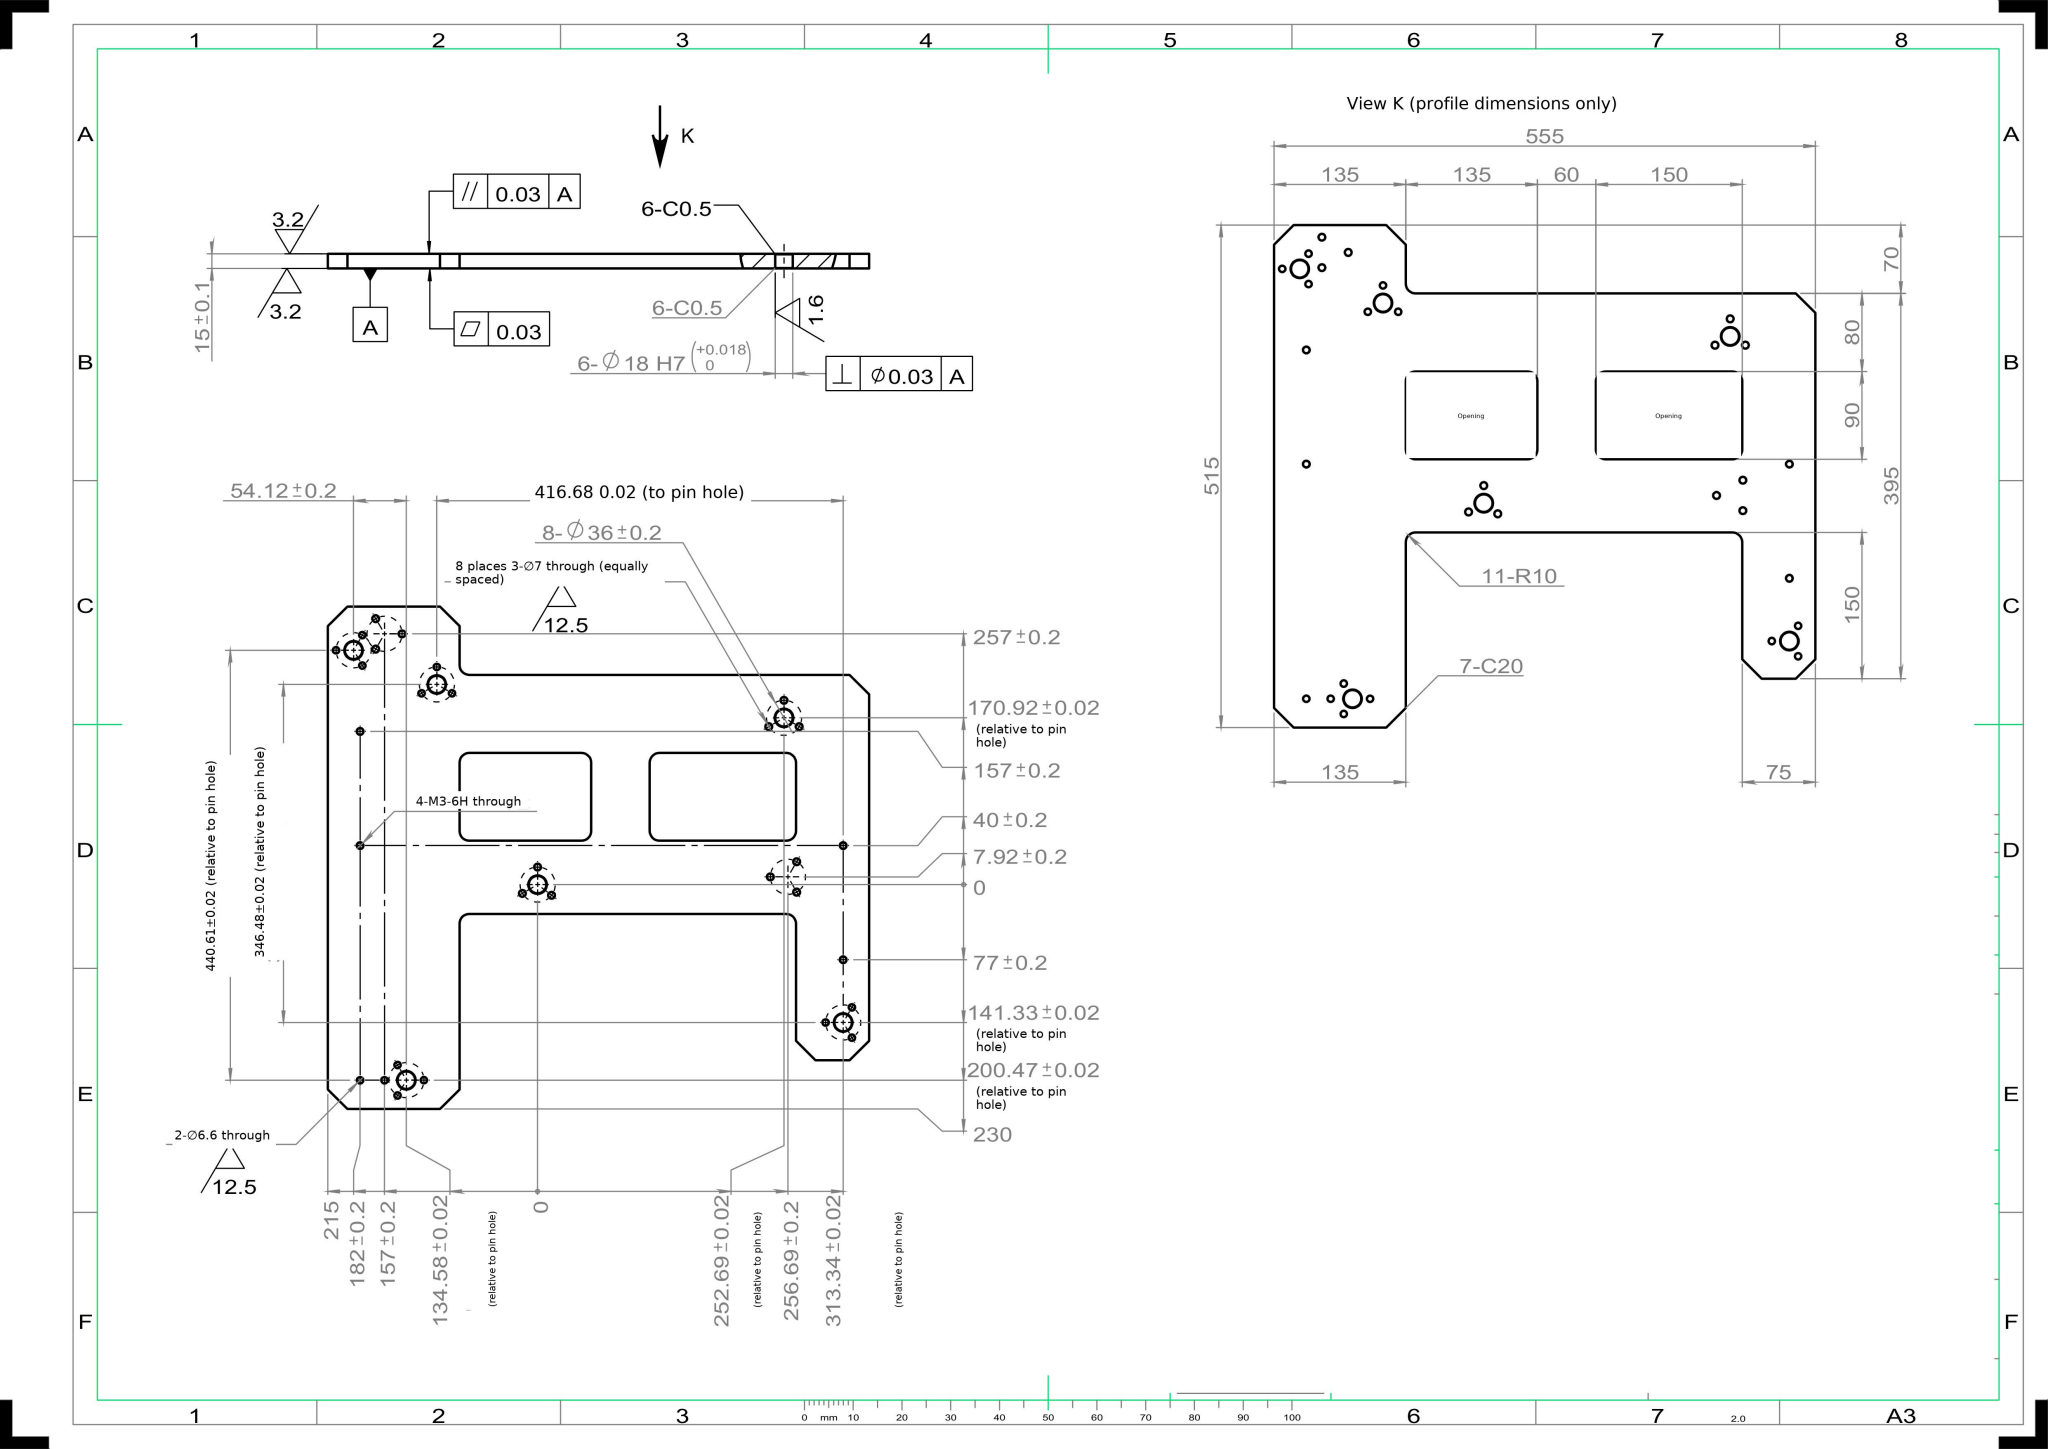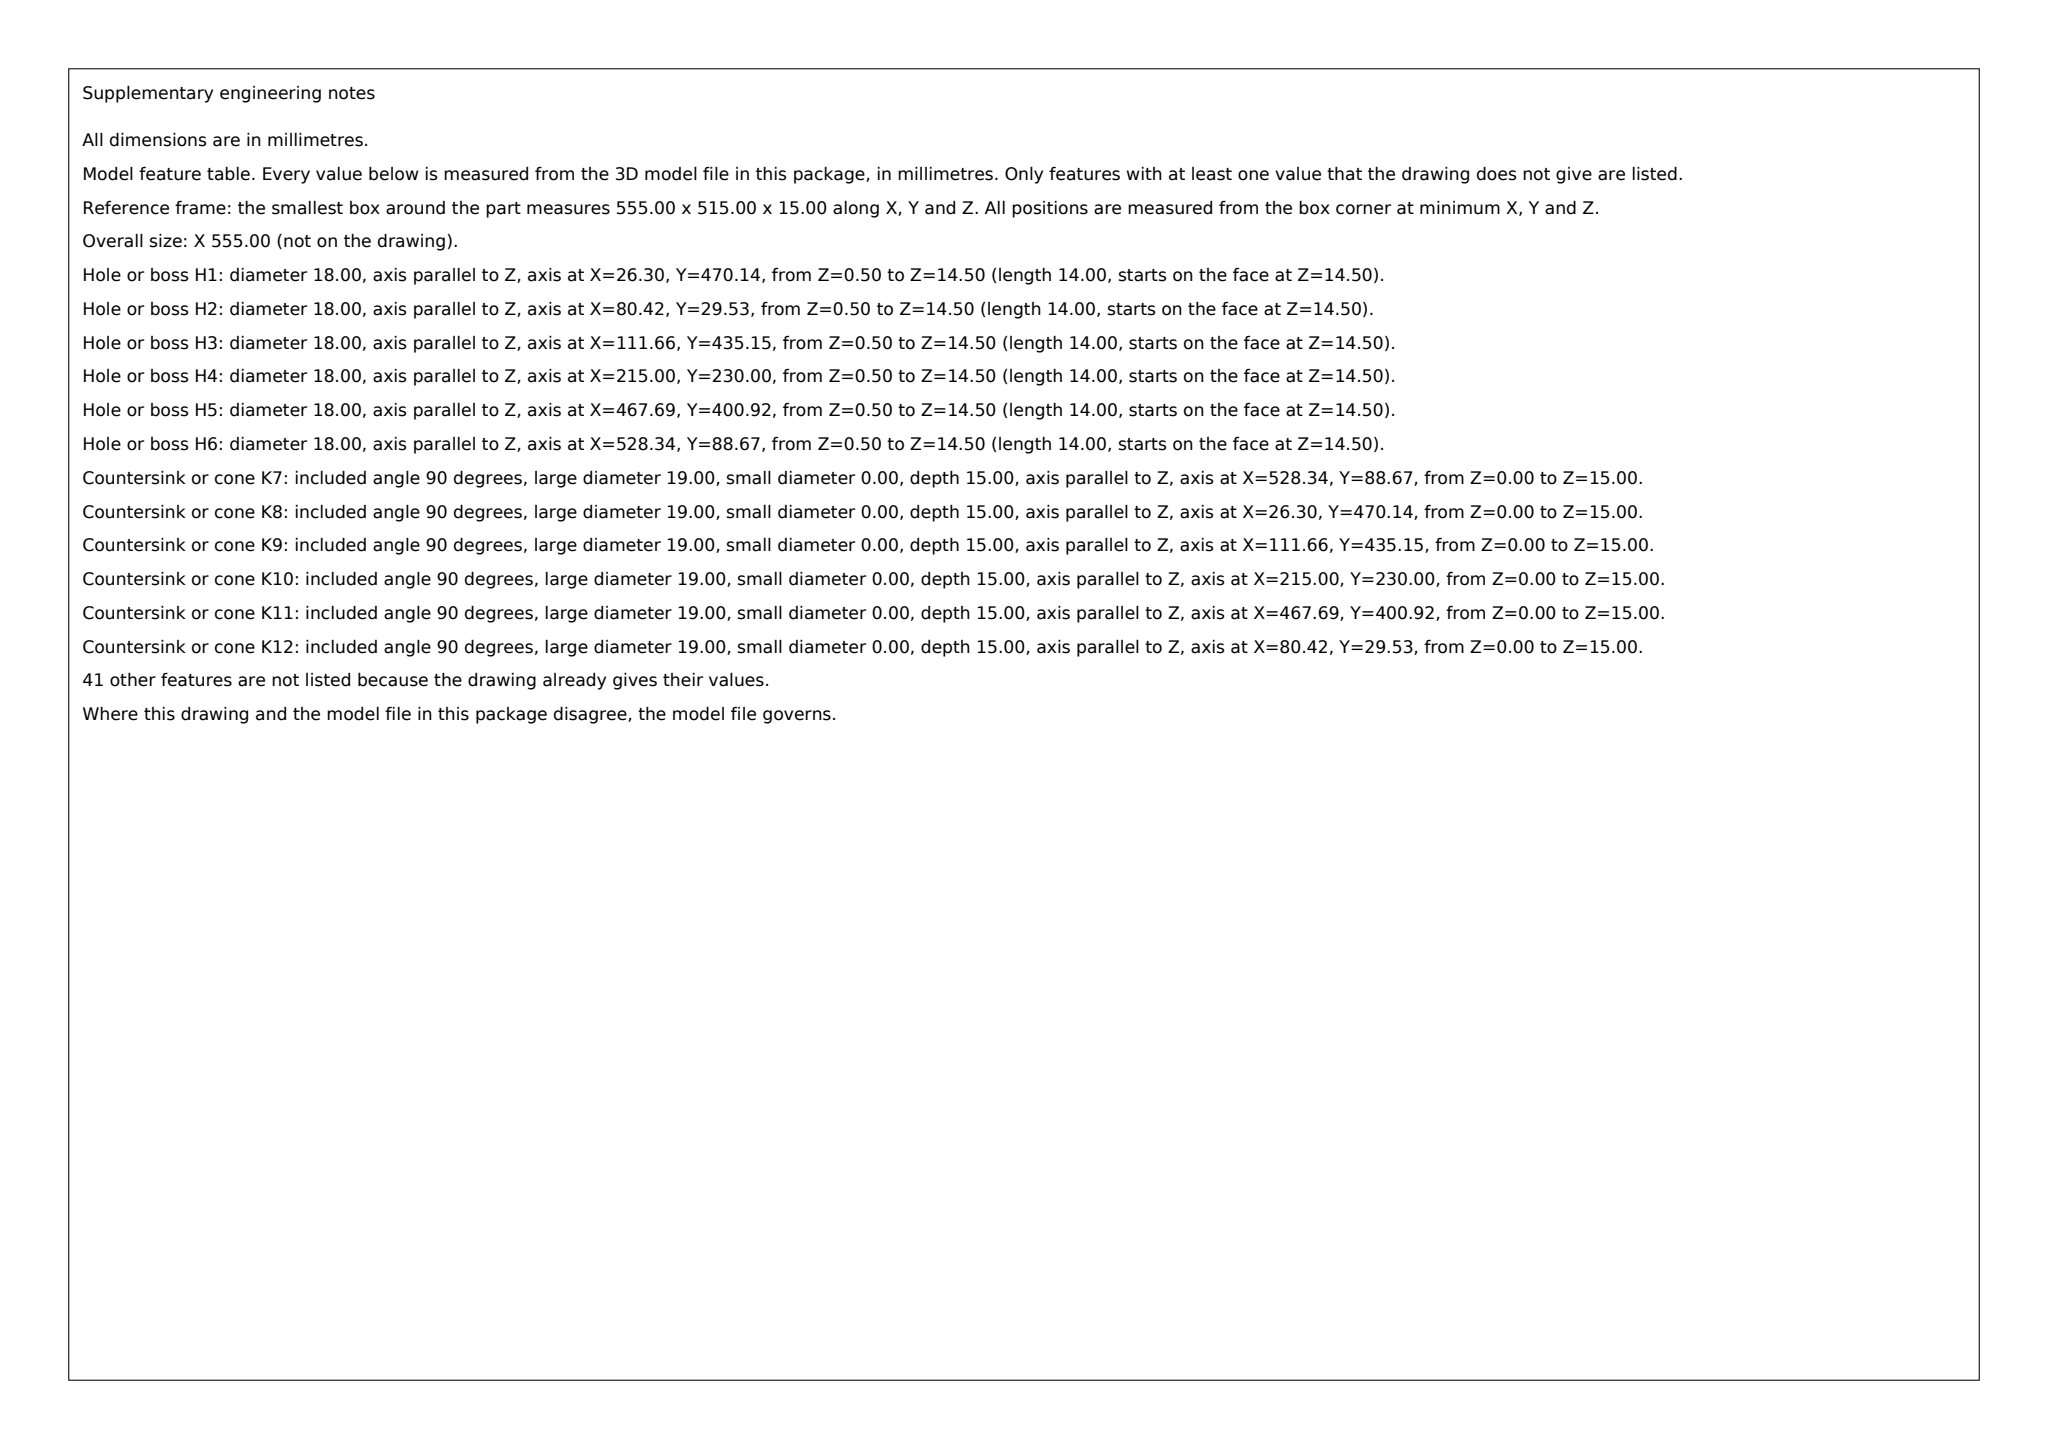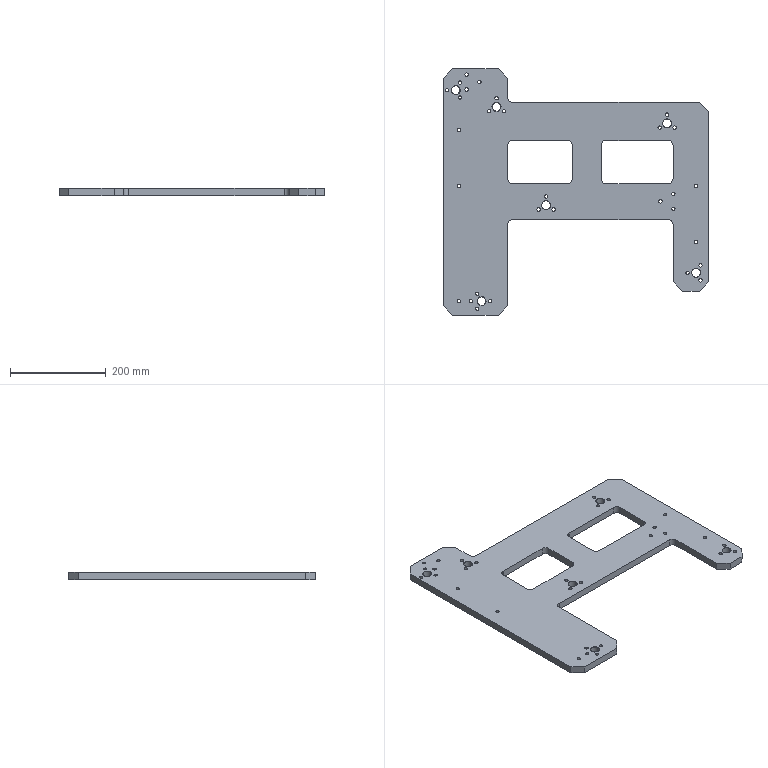Part | SolidWorks | mm | 1 solid | 134 faces | box 555 x 515 x 15 mm | volume 2312868 mm3 | cylinder 83 | plane 27 | cone 24 | commonest cylinder face diameters 7 x48 18 x12 20 x11 6.8 x8 6.6 x4